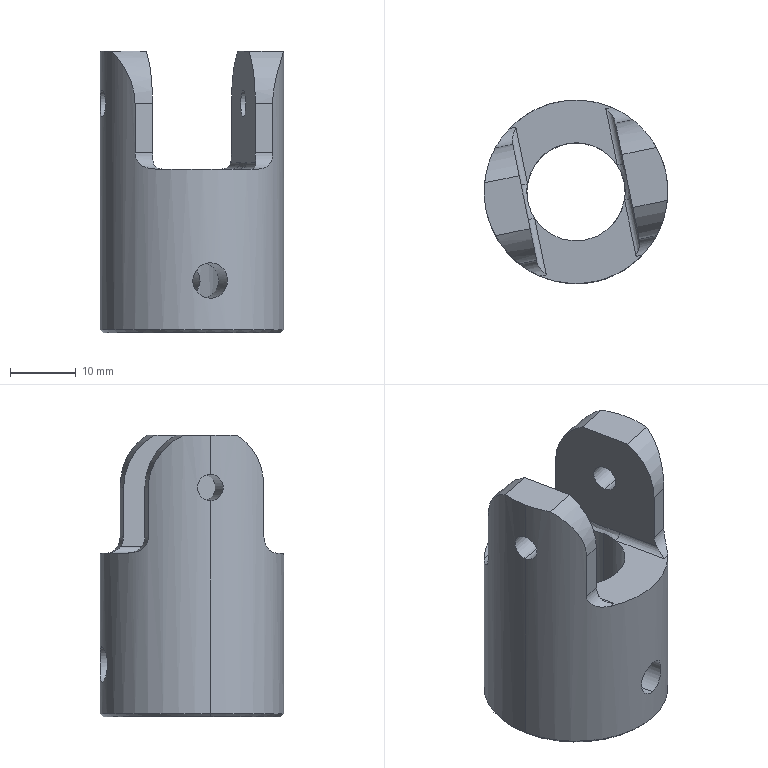Component | SolidWorks | DoubleFilmTransport-1_UniversalJointA-2 | 1 solid | 41 faces | volume 13583 mm3 | cylinder 24 | plane 11 | cone 4 | spline 2 | commonest cylinder face diameters 5.4 x4 4 x4 18 x4 4.978 x4 2 x4 28 x2 15 x2